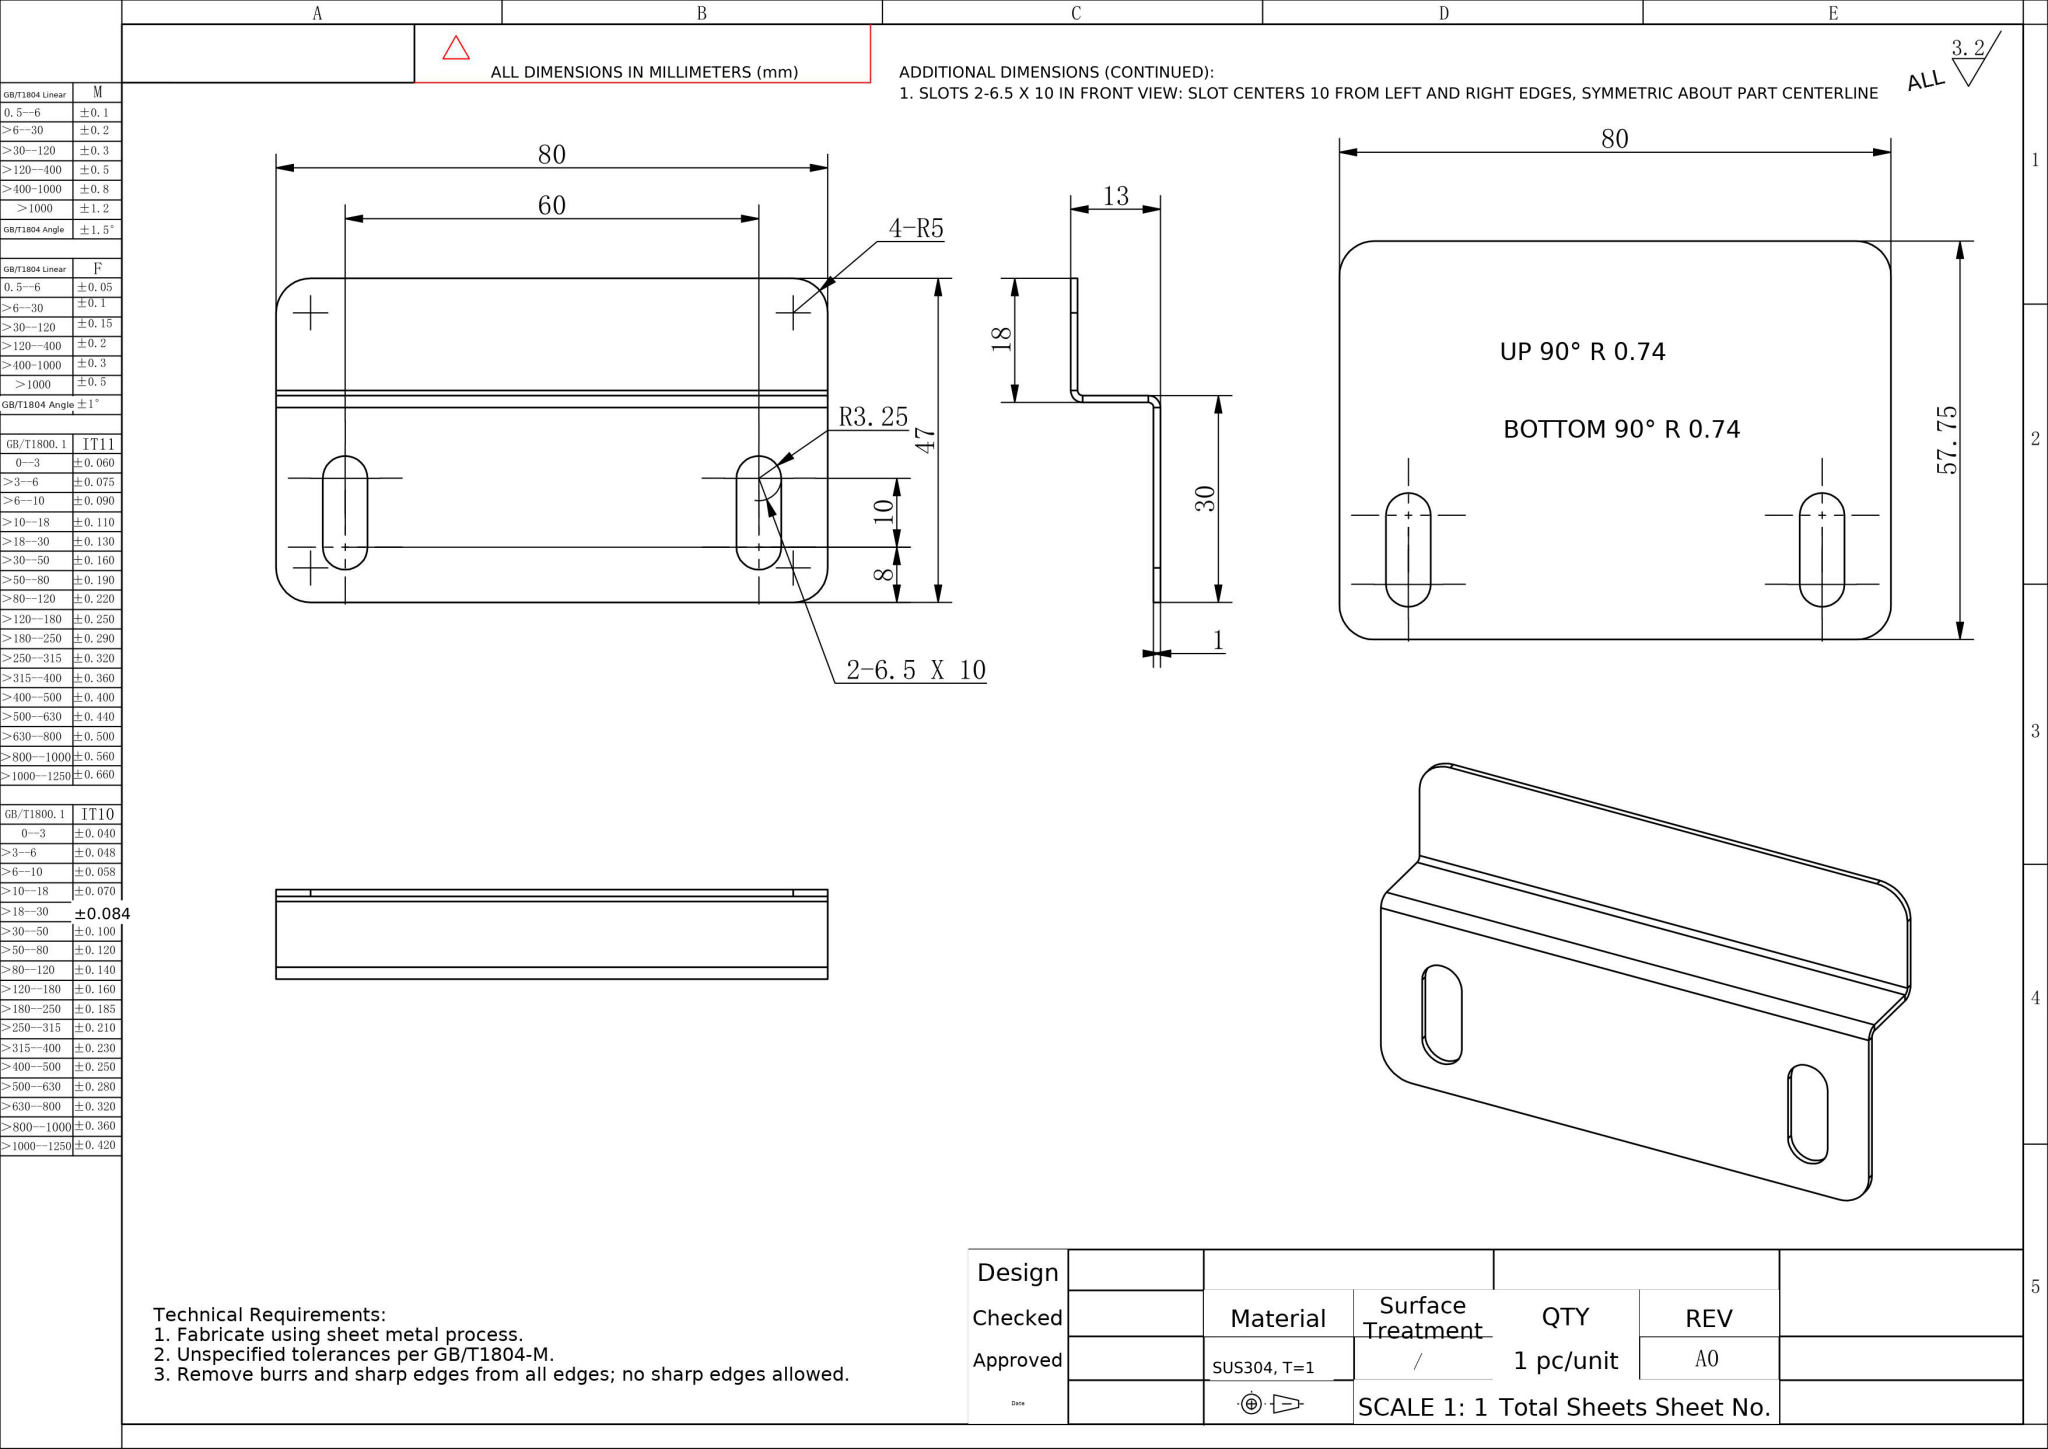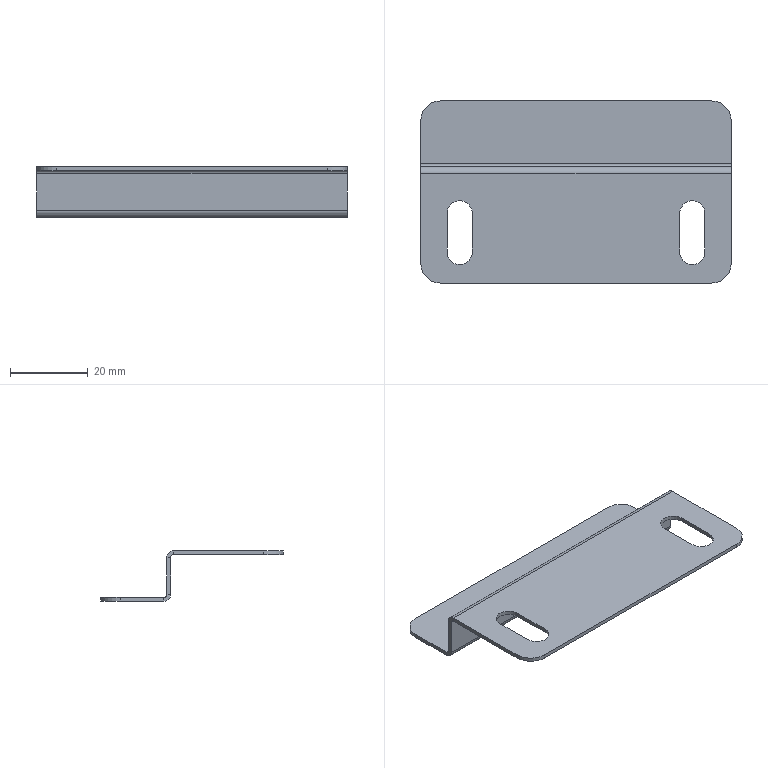Part | NX | mm | 1 solid | 34 faces | box 80 x 47 x 13 mm | volume 4417 mm3 | plane 22 | cylinder 12 | commonest cylinder face diameters 10 x4 6.5 x4 3.473 x2 1.473 x2
STEP:
#1=COLOUR_RGB('',0.7529,0.7529,0.7529);
#2=FILL_AREA_STYLE_COLOUR('',#1);
#3=FILL_AREA_STYLE('',(#2));
#4=SURFACE_STYLE_FILL_AREA(#3);
#5=SURFACE_SIDE_STYLE('',(#4));
#6=SURFACE_STYLE_USAGE(.BOTH.,#5);
#7=PRESENTATION_STYLE_ASSIGNMENT((#6));
#8=CARTESIAN_POINT('',(-40.,-9.737,12.));
#9=VERTEX_POINT('',#8);
#10=CARTESIAN_POINT('',(-40.,-33.,12.));
#11=VERTEX_POINT('',#10);
#12=CARTESIAN_POINT('',(-40.,-0.,12.));
#13=DIRECTION('',(0.,-1.,0.));
#14=VECTOR('',#13,1000.);
#15=LINE('',#12,#14);
#16=EDGE_CURVE('',#9,#11,#15,.T.);
#17=ORIENTED_EDGE('',*,*,#16,.T.);
#18=CARTESIAN_POINT('',(-35.,-38.,12.));
#19=VERTEX_POINT('',#18);
#20=CARTESIAN_POINT('',(-35.,-33.,12.));
#21=DIRECTION('',(0.,0.,1.));
#22=DIRECTION('',(-1.,0.,0.));
#23=AXIS2_PLACEMENT_3D('',#20,#21,#22);
#24=CIRCLE('',#23,5.);
#25=EDGE_CURVE('',#11,#19,#24,.T.);
#26=ORIENTED_EDGE('',*,*,#25,.T.);
#27=CARTESIAN_POINT('',(35.,-38.,12.));
#28=VERTEX_POINT('',#27);
#29=CARTESIAN_POINT('',(0.,-38.,12.));
#30=DIRECTION('',(1.,0.,0.));
#31=VECTOR('',#30,1000.);
#32=LINE('',#29,#31);
#33=EDGE_CURVE('',#19,#28,#32,.T.);
#34=ORIENTED_EDGE('',*,*,#33,.T.);
#35=CARTESIAN_POINT('',(40.,-33.,12.));
#36=VERTEX_POINT('',#35);
#37=CARTESIAN_POINT('',(35.,-33.,12.));
#38=DIRECTION('',(0.,0.,1.));
#39=DIRECTION('',(-1.,0.,0.));
#40=AXIS2_PLACEMENT_3D('',#37,#38,#39);
#41=CIRCLE('',#40,5.);
#42=EDGE_CURVE('',#28,#36,#41,.T.);
#43=ORIENTED_EDGE('',*,*,#42,.T.);
#44=CARTESIAN_POINT('',(40.,-9.737,12.));
#45=VERTEX_POINT('',#44);
#46=CARTESIAN_POINT('',(40.,0.,12.));
#47=DIRECTION('',(0.,1.,0.));
#48=VECTOR('',#47,1000.);
#49=LINE('',#46,#48);
#50=EDGE_CURVE('',#36,#45,#49,.T.);
#51=ORIENTED_EDGE('',*,*,#50,.T.);
#52=CARTESIAN_POINT('',(40.,-9.737,12.));
#53=DIRECTION('',(1.,0.,0.));
#54=VECTOR('',#53,1000.);
#55=LINE('',#52,#54);
#56=EDGE_CURVE('',#9,#45,#55,.T.);
#57=ORIENTED_EDGE('',*,*,#56,.F.);
#58=EDGE_LOOP('',(#17,#26,#34,#43,#51,#57));
#59=FACE_OUTER_BOUND('',#58,.T.);
#60=CARTESIAN_POINT('',(-33.25,-20.,12.));
#61=VERTEX_POINT('',#60);
#62=CARTESIAN_POINT('',(-33.25,-30.,12.));
#63=VERTEX_POINT('',#62);
#64=CARTESIAN_POINT('',(-33.25,-20.,12.));
#65=DIRECTION('',(0.,-1.,0.));
#66=VECTOR('',#65,1000.);
#67=LINE('',#64,#66);
#68=EDGE_CURVE('',#61,#63,#67,.T.);
#69=ORIENTED_EDGE('',*,*,#68,.F.);
#70=CARTESIAN_POINT('',(-26.75,-20.,12.));
#71=VERTEX_POINT('',#70);
#72=CARTESIAN_POINT('',(-30.,-20.,12.));
#73=DIRECTION('',(0.,0.,1.));
#74=DIRECTION('',(1.,0.,0.));
#75=AXIS2_PLACEMENT_3D('',#72,#73,#74);
#76=CIRCLE('',#75,3.25);
#77=EDGE_CURVE('',#71,#61,#76,.T.);
#78=ORIENTED_EDGE('',*,*,#77,.F.);
#79=CARTESIAN_POINT('',(-26.75,-30.,12.));
#80=VERTEX_POINT('',#79);
#81=CARTESIAN_POINT('',(-26.75,-20.,12.));
#82=DIRECTION('',(0.,1.,0.));
#83=VECTOR('',#82,1000.);
#84=LINE('',#81,#83);
#85=EDGE_CURVE('',#80,#71,#84,.T.);
#86=ORIENTED_EDGE('',*,*,#85,.F.);
#87=CARTESIAN_POINT('',(-30.,-30.,12.));
#88=DIRECTION('',(0.,0.,1.));
#89=DIRECTION('',(1.,0.,0.));
#90=AXIS2_PLACEMENT_3D('',#87,#88,#89);
#91=CIRCLE('',#90,3.25);
#92=EDGE_CURVE('',#63,#80,#91,.T.);
#93=ORIENTED_EDGE('',*,*,#92,.F.);
#94=EDGE_LOOP('',(#69,#78,#86,#93));
#95=FACE_BOUND('',#94,.T.);
#96=CARTESIAN_POINT('',(26.75,-20.,12.));
#97=VERTEX_POINT('',#96);
#98=CARTESIAN_POINT('',(33.25,-20.,12.));
#99=VERTEX_POINT('',#98);
#100=CARTESIAN_POINT('',(30.,-20.,12.));
#101=DIRECTION('',(-0.,-0.,-1.));
#102=DIRECTION('',(-1.,0.,0.));
#103=AXIS2_PLACEMENT_3D('',#100,#101,#102);
#104=CIRCLE('',#103,3.25);
#105=EDGE_CURVE('',#97,#99,#104,.T.);
#106=ORIENTED_EDGE('',*,*,#105,.T.);
#107=CARTESIAN_POINT('',(33.25,-30.,12.));
#108=VERTEX_POINT('',#107);
#109=CARTESIAN_POINT('',(33.25,-20.,12.));
#110=DIRECTION('',(-0.,-1.,0.));
#111=VECTOR('',#110,1000.);
#112=LINE('',#109,#111);
#113=EDGE_CURVE('',#99,#108,#112,.T.);
#114=ORIENTED_EDGE('',*,*,#113,.T.);
#115=CARTESIAN_POINT('',(26.75,-30.,12.));
#116=VERTEX_POINT('',#115);
#117=CARTESIAN_POINT('',(30.,-30.,12.));
#118=DIRECTION('',(-0.,-0.,-1.));
#119=DIRECTION('',(-1.,0.,0.));
#120=AXIS2_PLACEMENT_3D('',#117,#118,#119);
#121=CIRCLE('',#120,3.25);
#122=EDGE_CURVE('',#108,#116,#121,.T.);
#123=ORIENTED_EDGE('',*,*,#122,.T.);
#124=CARTESIAN_POINT('',(26.75,-20.,12.));
#125=DIRECTION('',(-0.,1.,0.));
#126=VECTOR('',#125,1000.);
#127=LINE('',#124,#126);
#128=EDGE_CURVE('',#116,#97,#127,.T.);
#129=ORIENTED_EDGE('',*,*,#128,.T.);
#130=EDGE_LOOP('',(#106,#114,#123,#129));
#131=FACE_BOUND('',#130,.T.);
#132=CARTESIAN_POINT('',(0.,0.,12.));
#133=DIRECTION('',(0.,0.,-1.));
#134=DIRECTION('',(-1.,0.,0.));
#135=AXIS2_PLACEMENT_3D('',#132,#133,#134);
#136=PLANE('',#135);
#137=ADVANCED_FACE('',(#59,#95,#131),#136,.F.);
#138=CARTESIAN_POINT('',(-33.25,-20.,11.));
#139=VERTEX_POINT('',#138);
#140=CARTESIAN_POINT('',(-26.75,-20.,11.));
#141=VERTEX_POINT('',#140);
#142=CARTESIAN_POINT('',(-30.,-20.,11.));
#143=DIRECTION('',(0.,0.,-1.));
#144=DIRECTION('',(-1.,0.,0.));
#145=AXIS2_PLACEMENT_3D('',#142,#143,#144);
#146=CIRCLE('',#145,3.25);
#147=EDGE_CURVE('',#139,#141,#146,.T.);
#148=ORIENTED_EDGE('',*,*,#147,.F.);
#149=CARTESIAN_POINT('',(-33.25,-30.,11.));
#150=VERTEX_POINT('',#149);
#151=CARTESIAN_POINT('',(-33.25,-0.,11.));
#152=DIRECTION('',(-0.,1.,0.));
#153=VECTOR('',#152,1000.);
#154=LINE('',#151,#153);
#155=EDGE_CURVE('',#150,#139,#154,.T.);
#156=ORIENTED_EDGE('',*,*,#155,.F.);
#157=CARTESIAN_POINT('',(-26.75,-30.,11.));
#158=VERTEX_POINT('',#157);
#159=CARTESIAN_POINT('',(-30.,-30.,11.));
#160=DIRECTION('',(0.,0.,-1.));
#161=DIRECTION('',(-1.,0.,0.));
#162=AXIS2_PLACEMENT_3D('',#159,#160,#161);
#163=CIRCLE('',#162,3.25);
#164=EDGE_CURVE('',#158,#150,#163,.T.);
#165=ORIENTED_EDGE('',*,*,#164,.F.);
#166=CARTESIAN_POINT('',(-26.75,0.,11.));
#167=DIRECTION('',(0.,-1.,0.));
#168=VECTOR('',#167,1000.);
#169=LINE('',#166,#168);
#170=EDGE_CURVE('',#141,#158,#169,.T.);
#171=ORIENTED_EDGE('',*,*,#170,.F.);
#172=EDGE_LOOP('',(#148,#156,#165,#171));
#173=FACE_BOUND('',#172,.T.);
#174=CARTESIAN_POINT('',(-35.,-38.,11.));
#175=VERTEX_POINT('',#174);
#176=CARTESIAN_POINT('',(35.,-38.,11.));
#177=VERTEX_POINT('',#176);
#178=CARTESIAN_POINT('',(40.,-38.,11.));
#179=DIRECTION('',(1.,0.,0.));
#180=VECTOR('',#179,1000.);
#181=LINE('',#178,#180);
#182=EDGE_CURVE('',#175,#177,#181,.T.);
#183=ORIENTED_EDGE('',*,*,#182,.F.);
#184=CARTESIAN_POINT('',(-40.,-33.,11.));
#185=VERTEX_POINT('',#184);
#186=CARTESIAN_POINT('',(-35.,-33.,11.));
#187=DIRECTION('',(0.,0.,-1.));
#188=DIRECTION('',(-1.,0.,0.));
#189=AXIS2_PLACEMENT_3D('',#186,#187,#188);
#190=CIRCLE('',#189,5.);
#191=EDGE_CURVE('',#175,#185,#190,.T.);
#192=ORIENTED_EDGE('',*,*,#191,.T.);
#193=CARTESIAN_POINT('',(-40.,-9.737,11.));
#194=VERTEX_POINT('',#193);
#195=CARTESIAN_POINT('',(-40.,-38.,11.));
#196=DIRECTION('',(0.,-1.,0.));
#197=VECTOR('',#196,1000.);
#198=LINE('',#195,#197);
#199=EDGE_CURVE('',#194,#185,#198,.T.);
#200=ORIENTED_EDGE('',*,*,#199,.F.);
#201=CARTESIAN_POINT('',(40.,-9.737,11.));
#202=VERTEX_POINT('',#201);
#203=CARTESIAN_POINT('',(40.,-9.737,11.));
#204=DIRECTION('',(-1.,0.,0.));
#205=VECTOR('',#204,1000.);
#206=LINE('',#203,#205);
#207=EDGE_CURVE('',#202,#194,#206,.T.);
#208=ORIENTED_EDGE('',*,*,#207,.F.);
#209=CARTESIAN_POINT('',(40.,-33.,11.));
#210=VERTEX_POINT('',#209);
#211=CARTESIAN_POINT('',(40.,-9.,11.));
#212=DIRECTION('',(0.,1.,0.));
#213=VECTOR('',#212,1000.);
#214=LINE('',#211,#213);
#215=EDGE_CURVE('',#210,#202,#214,.T.);
#216=ORIENTED_EDGE('',*,*,#215,.F.);
#217=CARTESIAN_POINT('',(35.,-33.,11.));
#218=DIRECTION('',(0.,0.,-1.));
#219=DIRECTION('',(-1.,0.,0.));
#220=AXIS2_PLACEMENT_3D('',#217,#218,#219);
#221=CIRCLE('',#220,5.);
#222=EDGE_CURVE('',#210,#177,#221,.T.);
#223=ORIENTED_EDGE('',*,*,#222,.T.);
#224=EDGE_LOOP('',(#183,#192,#200,#208,#216,#223));
#225=FACE_OUTER_BOUND('',#224,.T.);
#226=CARTESIAN_POINT('',(33.25,-30.,11.));
#227=VERTEX_POINT('',#226);
#228=CARTESIAN_POINT('',(33.25,-20.,11.));
#229=VERTEX_POINT('',#228);
#230=CARTESIAN_POINT('',(33.25,-0.,11.));
#231=DIRECTION('',(0.,1.,0.));
#232=VECTOR('',#231,1000.);
#233=LINE('',#230,#232);
#234=EDGE_CURVE('',#227,#229,#233,.T.);
#235=ORIENTED_EDGE('',*,*,#234,.T.);
#236=CARTESIAN_POINT('',(26.75,-20.,11.));
#237=VERTEX_POINT('',#236);
#238=CARTESIAN_POINT('',(30.,-20.,11.));
#239=DIRECTION('',(0.,0.,1.));
#240=DIRECTION('',(-1.,0.,0.));
#241=AXIS2_PLACEMENT_3D('',#238,#239,#240);
#242=CIRCLE('',#241,3.25);
#243=EDGE_CURVE('',#229,#237,#242,.T.);
#244=ORIENTED_EDGE('',*,*,#243,.T.);
#245=CARTESIAN_POINT('',(26.75,-30.,11.));
#246=VERTEX_POINT('',#245);
#247=CARTESIAN_POINT('',(26.75,0.,11.));
#248=DIRECTION('',(0.,-1.,0.));
#249=VECTOR('',#248,1000.);
#250=LINE('',#247,#249);
#251=EDGE_CURVE('',#237,#246,#250,.T.);
#252=ORIENTED_EDGE('',*,*,#251,.T.);
#253=CARTESIAN_POINT('',(30.,-30.,11.));
#254=DIRECTION('',(0.,0.,1.));
#255=DIRECTION('',(-1.,0.,0.));
#256=AXIS2_PLACEMENT_3D('',#253,#254,#255);
#257=CIRCLE('',#256,3.25);
#258=EDGE_CURVE('',#246,#227,#257,.T.);
#259=ORIENTED_EDGE('',*,*,#258,.T.);
#260=EDGE_LOOP('',(#235,#244,#252,#259));
#261=FACE_BOUND('',#260,.T.);
#262=CARTESIAN_POINT('',(0.,0.,11.));
#263=DIRECTION('',(0.,0.,-1.));
#264=DIRECTION('',(-1.,0.,0.));
#265=AXIS2_PLACEMENT_3D('',#262,#263,#264);
#266=PLANE('',#265);
#267=ADVANCED_FACE('',(#173,#225,#261),#266,.T.);
#268=CARTESIAN_POINT('',(-40.,-9.,10.263));
#269=VERTEX_POINT('',#268);
#270=CARTESIAN_POINT('',(-40.,-8.,10.263));
#271=VERTEX_POINT('',#270);
#272=CARTESIAN_POINT('',(-40.,-9.,10.263));
#273=DIRECTION('',(-0.,1.,-0.));
#274=VECTOR('',#273,1000.);
#275=LINE('',#272,#274);
#276=EDGE_CURVE('',#269,#271,#275,.T.);
#277=ORIENTED_EDGE('',*,*,#276,.T.);
#278=CARTESIAN_POINT('',(-40.,-8.,0.7366));
#279=VERTEX_POINT('',#278);
#280=CARTESIAN_POINT('',(-40.,-8.,-0.));
#281=DIRECTION('',(0.,0.,-1.));
#282=VECTOR('',#281,1000.);
#283=LINE('',#280,#282);
#284=EDGE_CURVE('',#271,#279,#283,.T.);
#285=ORIENTED_EDGE('',*,*,#284,.T.);
#286=CARTESIAN_POINT('',(-40.,-9.,0.7366));
#287=VERTEX_POINT('',#286);
#288=CARTESIAN_POINT('',(-40.,-9.,0.7366));
#289=DIRECTION('',(0.,-1.,-0.));
#290=VECTOR('',#289,1000.);
#291=LINE('',#288,#290);
#292=EDGE_CURVE('',#279,#287,#291,.T.);
#293=ORIENTED_EDGE('',*,*,#292,.T.);
#294=CARTESIAN_POINT('',(-40.,-9.,-0.));
#295=DIRECTION('',(0.,0.,-1.));
#296=VECTOR('',#295,1000.);
#297=LINE('',#294,#296);
#298=EDGE_CURVE('',#269,#287,#297,.T.);
#299=ORIENTED_EDGE('',*,*,#298,.F.);
#300=EDGE_LOOP('',(#277,#285,#293,#299));
#301=FACE_OUTER_BOUND('',#300,.T.);
#302=CARTESIAN_POINT('',(-40.,-9.,-0.));
#303=DIRECTION('',(1.,0.,0.));
#304=DIRECTION('',(0.,0.,-1.));
#305=AXIS2_PLACEMENT_3D('',#302,#303,#304);
#306=PLANE('',#305);
#307=ADVANCED_FACE('',(#301),#306,.F.);
#308=CARTESIAN_POINT('',(40.,-9.,10.263));
#309=VERTEX_POINT('',#308);
#310=CARTESIAN_POINT('',(40.,-8.,10.263));
#311=VERTEX_POINT('',#310);
#312=CARTESIAN_POINT('',(40.,-9.,10.263));
#313=DIRECTION('',(0.,1.,-0.));
#314=VECTOR('',#313,1000.);
#315=LINE('',#312,#314);
#316=EDGE_CURVE('',#309,#311,#315,.T.);
#317=ORIENTED_EDGE('',*,*,#316,.F.);
#318=CARTESIAN_POINT('',(40.,-9.,0.7366));
#319=VERTEX_POINT('',#318);
#320=CARTESIAN_POINT('',(40.,-9.,-0.));
#321=DIRECTION('',(0.,-0.,1.));
#322=VECTOR('',#321,1000.);
#323=LINE('',#320,#322);
#324=EDGE_CURVE('',#319,#309,#323,.T.);
#325=ORIENTED_EDGE('',*,*,#324,.F.);
#326=CARTESIAN_POINT('',(40.,-8.,0.7366));
#327=VERTEX_POINT('',#326);
#328=CARTESIAN_POINT('',(40.,-8.,0.7366));
#329=DIRECTION('',(0.,-1.,-0.));
#330=VECTOR('',#329,1000.);
#331=LINE('',#328,#330);
#332=EDGE_CURVE('',#327,#319,#331,.T.);
#333=ORIENTED_EDGE('',*,*,#332,.F.);
#334=CARTESIAN_POINT('',(40.,-8.,12.));
#335=DIRECTION('',(0.,-0.,1.));
#336=VECTOR('',#335,1000.);
#337=LINE('',#334,#336);
#338=EDGE_CURVE('',#327,#311,#337,.T.);
#339=ORIENTED_EDGE('',*,*,#338,.T.);
#340=EDGE_LOOP('',(#317,#325,#333,#339));
#341=FACE_OUTER_BOUND('',#340,.T.);
#342=CARTESIAN_POINT('',(40.,-9.,12.));
#343=DIRECTION('',(-1.,-0.,0.));
#344=DIRECTION('',(0.,0.,1.));
#345=AXIS2_PLACEMENT_3D('',#342,#343,#344);
#346=PLANE('',#345);
#347=ADVANCED_FACE('',(#341),#346,.F.);
#348=CARTESIAN_POINT('',(-40.,-9.,10.263));
#349=DIRECTION('',(1.,0.,-0.));
#350=VECTOR('',#349,1000.);
#351=LINE('',#348,#350);
#352=EDGE_CURVE('',#269,#309,#351,.T.);
#353=ORIENTED_EDGE('',*,*,#352,.F.);
#354=ORIENTED_EDGE('',*,*,#298,.T.);
#355=CARTESIAN_POINT('',(-40.,-9.,0.7366));
#356=DIRECTION('',(-1.,0.,0.));
#357=VECTOR('',#356,1000.);
#358=LINE('',#355,#357);
#359=EDGE_CURVE('',#319,#287,#358,.T.);
#360=ORIENTED_EDGE('',*,*,#359,.F.);
#361=ORIENTED_EDGE('',*,*,#324,.T.);
#362=EDGE_LOOP('',(#353,#354,#360,#361));
#363=FACE_OUTER_BOUND('',#362,.T.);
#364=CARTESIAN_POINT('',(0.,-9.,-0.));
#365=DIRECTION('',(0.,1.,0.));
#366=DIRECTION('',(0.,-0.,1.));
#367=AXIS2_PLACEMENT_3D('',#364,#365,#366);
#368=PLANE('',#367);
#369=ADVANCED_FACE('',(#363),#368,.F.);
#370=ORIENTED_EDGE('',*,*,#284,.F.);
#371=CARTESIAN_POINT('',(-40.,-8.,10.263));
#372=DIRECTION('',(1.,0.,-0.));
#373=VECTOR('',#372,1000.);
#374=LINE('',#371,#373);
#375=EDGE_CURVE('',#271,#311,#374,.T.);
#376=ORIENTED_EDGE('',*,*,#375,.T.);
#377=ORIENTED_EDGE('',*,*,#338,.F.);
#378=CARTESIAN_POINT('',(-40.,-8.,0.7366));
#379=DIRECTION('',(1.,0.,0.));
#380=VECTOR('',#379,1000.);
#381=LINE('',#378,#380);
#382=EDGE_CURVE('',#279,#327,#381,.T.);
#383=ORIENTED_EDGE('',*,*,#382,.F.);
#384=EDGE_LOOP('',(#370,#376,#377,#383));
#385=FACE_OUTER_BOUND('',#384,.T.);
#386=CARTESIAN_POINT('',(0.,-8.,-0.));
#387=DIRECTION('',(0.,1.,0.));
#388=DIRECTION('',(0.,-0.,1.));
#389=AXIS2_PLACEMENT_3D('',#386,#387,#388);
#390=PLANE('',#389);
#391=ADVANCED_FACE('',(#385),#390,.T.);
#392=CARTESIAN_POINT('',(40.,-7.263,-1.));
#393=VERTEX_POINT('',#392);
#394=CARTESIAN_POINT('',(40.,4.,-1.));
#395=VERTEX_POINT('',#394);
#396=CARTESIAN_POINT('',(40.,9.,-1.));
#397=DIRECTION('',(0.,1.,0.));
#398=VECTOR('',#397,1000.);
#399=LINE('',#396,#398);
#400=EDGE_CURVE('',#393,#395,#399,.T.);
#401=ORIENTED_EDGE('',*,*,#400,.T.);
#402=CARTESIAN_POINT('',(40.,4.,0.));
#403=VERTEX_POINT('',#402);
#404=CARTESIAN_POINT('',(40.,4.,-1.));
#405=DIRECTION('',(0.,0.,1.));
#406=VECTOR('',#405,1000.);
#407=LINE('',#404,#406);
#408=EDGE_CURVE('',#395,#403,#407,.T.);
#409=ORIENTED_EDGE('',*,*,#408,.T.);
#410=CARTESIAN_POINT('',(40.,-7.263,0.));
#411=VERTEX_POINT('',#410);
#412=CARTESIAN_POINT('',(40.,9.,0.));
#413=DIRECTION('',(0.,1.,0.));
#414=VECTOR('',#413,1000.);
#415=LINE('',#412,#414);
#416=EDGE_CURVE('',#411,#403,#415,.T.);
#417=ORIENTED_EDGE('',*,*,#416,.F.);
#418=CARTESIAN_POINT('',(40.,-7.263,-0.));
#419=DIRECTION('',(0.,0.,-1.));
#420=VECTOR('',#419,1000.);
#421=LINE('',#418,#420);
#422=EDGE_CURVE('',#411,#393,#421,.T.);
#423=ORIENTED_EDGE('',*,*,#422,.T.);
#424=EDGE_LOOP('',(#401,#409,#417,#423));
#425=FACE_OUTER_BOUND('',#424,.T.);
#426=CARTESIAN_POINT('',(40.,9.,-1.));
#427=DIRECTION('',(1.,0.,0.));
#428=DIRECTION('',(0.,0.,-1.));
#429=AXIS2_PLACEMENT_3D('',#426,#427,#428);
#430=PLANE('',#429);
#431=ADVANCED_FACE('',(#425),#430,.T.);
#432=CARTESIAN_POINT('',(35.,9.,-1.));
#433=VERTEX_POINT('',#432);
#434=CARTESIAN_POINT('',(-35.,9.,-1.));
#435=VERTEX_POINT('',#434);
#436=CARTESIAN_POINT('',(-40.,9.,-1.));
#437=DIRECTION('',(-1.,0.,0.));
#438=VECTOR('',#437,1000.);
#439=LINE('',#436,#438);
#440=EDGE_CURVE('',#433,#435,#439,.T.);
#441=ORIENTED_EDGE('',*,*,#440,.F.);
#442=CARTESIAN_POINT('',(35.,4.,-1.));
#443=DIRECTION('',(0.,0.,-1.));
#444=DIRECTION('',(1.,0.,0.));
#445=AXIS2_PLACEMENT_3D('',#442,#443,#444);
#446=CIRCLE('',#445,5.);
#447=EDGE_CURVE('',#433,#395,#446,.T.);
#448=ORIENTED_EDGE('',*,*,#447,.T.);
#449=ORIENTED_EDGE('',*,*,#400,.F.);
#450=CARTESIAN_POINT('',(-40.,-7.263,-1.));
#451=VERTEX_POINT('',#450);
#452=CARTESIAN_POINT('',(40.,-7.263,-1.));
#453=DIRECTION('',(-1.,0.,0.));
#454=VECTOR('',#453,1000.);
#455=LINE('',#452,#454);
#456=EDGE_CURVE('',#393,#451,#455,.T.);
#457=ORIENTED_EDGE('',*,*,#456,.T.);
#458=CARTESIAN_POINT('',(-40.,4.,-1.));
#459=VERTEX_POINT('',#458);
#460=CARTESIAN_POINT('',(-40.,9.,-1.));
#461=DIRECTION('',(0.,-1.,0.));
#462=VECTOR('',#461,1000.);
#463=LINE('',#460,#462);
#464=EDGE_CURVE('',#459,#451,#463,.T.);
#465=ORIENTED_EDGE('',*,*,#464,.F.);
#466=CARTESIAN_POINT('',(-35.,4.,-1.));
#467=DIRECTION('',(0.,0.,-1.));
#468=DIRECTION('',(1.,0.,0.));
#469=AXIS2_PLACEMENT_3D('',#466,#467,#468);
#470=CIRCLE('',#469,5.);
#471=EDGE_CURVE('',#459,#435,#470,.T.);
#472=ORIENTED_EDGE('',*,*,#471,.T.);
#473=EDGE_LOOP('',(#441,#448,#449,#457,#465,#472));
#474=FACE_OUTER_BOUND('',#473,.T.);
#475=CARTESIAN_POINT('',(0.,0.,-1.));
#476=DIRECTION('',(0.,0.,1.));
#477=DIRECTION('',(1.,0.,0.));
#478=AXIS2_PLACEMENT_3D('',#475,#476,#477);
#479=PLANE('',#478);
#480=ADVANCED_FACE('',(#474),#479,.F.);
#481=ORIENTED_EDGE('',*,*,#416,.T.);
#482=CARTESIAN_POINT('',(35.,9.,0.));
#483=VERTEX_POINT('',#482);
#484=CARTESIAN_POINT('',(35.,4.,0.));
#485=DIRECTION('',(0.,0.,1.));
#486=DIRECTION('',(1.,0.,0.));
#487=AXIS2_PLACEMENT_3D('',#484,#485,#486);
#488=CIRCLE('',#487,5.);
#489=EDGE_CURVE('',#403,#483,#488,.T.);
#490=ORIENTED_EDGE('',*,*,#489,.T.);
#491=CARTESIAN_POINT('',(-35.,9.,0.));
#492=VERTEX_POINT('',#491);
#493=CARTESIAN_POINT('',(-40.,9.,0.));
#494=DIRECTION('',(-1.,0.,0.));
#495=VECTOR('',#494,1000.);
#496=LINE('',#493,#495);
#497=EDGE_CURVE('',#483,#492,#496,.T.);
#498=ORIENTED_EDGE('',*,*,#497,.T.);
#499=CARTESIAN_POINT('',(-40.,4.,0.));
#500=VERTEX_POINT('',#499);
#501=CARTESIAN_POINT('',(-35.,4.,0.));
#502=DIRECTION('',(0.,0.,1.));
#503=DIRECTION('',(1.,0.,0.));
#504=AXIS2_PLACEMENT_3D('',#501,#502,#503);
#505=CIRCLE('',#504,5.);
#506=EDGE_CURVE('',#492,#500,#505,.T.);
#507=ORIENTED_EDGE('',*,*,#506,.T.);
#508=CARTESIAN_POINT('',(-40.,-7.263,-0.));
#509=VERTEX_POINT('',#508);
#510=CARTESIAN_POINT('',(-40.,9.,0.));
#511=DIRECTION('',(0.,-1.,0.));
#512=VECTOR('',#511,1000.);
#513=LINE('',#510,#512);
#514=EDGE_CURVE('',#500,#509,#513,.T.);
#515=ORIENTED_EDGE('',*,*,#514,.T.);
#516=CARTESIAN_POINT('',(40.,-7.263,-0.));
#517=DIRECTION('',(-1.,0.,0.));
#518=VECTOR('',#517,1000.);
#519=LINE('',#516,#518);
#520=EDGE_CURVE('',#411,#509,#519,.T.);
#521=ORIENTED_EDGE('',*,*,#520,.F.);
#522=EDGE_LOOP('',(#481,#490,#498,#507,#515,#521));
#523=FACE_OUTER_BOUND('',#522,.T.);
#524=CARTESIAN_POINT('',(0.,0.,0.));
#525=DIRECTION('',(0.,0.,1.));
#526=DIRECTION('',(1.,0.,0.));
#527=AXIS2_PLACEMENT_3D('',#524,#525,#526);
#528=PLANE('',#527);
#529=ADVANCED_FACE('',(#523),#528,.T.);
#530=ORIENTED_EDGE('',*,*,#514,.F.);
#531=CARTESIAN_POINT('',(-40.,4.,-1.));
#532=DIRECTION('',(0.,0.,-1.));
#533=VECTOR('',#532,1000.);
#534=LINE('',#531,#533);
#535=EDGE_CURVE('',#500,#459,#534,.T.);
#536=ORIENTED_EDGE('',*,*,#535,.T.);
#537=ORIENTED_EDGE('',*,*,#464,.T.);
#538=CARTESIAN_POINT('',(-40.,-7.263,-0.));
#539=DIRECTION('',(0.,0.,-1.));
#540=VECTOR('',#539,1000.);
#541=LINE('',#538,#540);
#542=EDGE_CURVE('',#509,#451,#541,.T.);
#543=ORIENTED_EDGE('',*,*,#542,.F.);
#544=EDGE_LOOP('',(#530,#536,#537,#543));
#545=FACE_OUTER_BOUND('',#544,.T.);
#546=CARTESIAN_POINT('',(-40.,9.,-1.));
#547=DIRECTION('',(-1.,0.,0.));
#548=DIRECTION('',(0.,0.,1.));
#549=AXIS2_PLACEMENT_3D('',#546,#547,#548);
#550=PLANE('',#549);
#551=ADVANCED_FACE('',(#545),#550,.T.);
#552=ORIENTED_EDGE('',*,*,#497,.F.);
#553=CARTESIAN_POINT('',(35.,9.,-1.));
#554=DIRECTION('',(0.,0.,-1.));
#555=VECTOR('',#554,1000.);
#556=LINE('',#553,#555);
#557=EDGE_CURVE('',#483,#433,#556,.T.);
#558=ORIENTED_EDGE('',*,*,#557,.T.);
#559=ORIENTED_EDGE('',*,*,#440,.T.);
#560=CARTESIAN_POINT('',(-35.,9.,-1.));
#561=DIRECTION('',(0.,0.,1.));
#562=VECTOR('',#561,1000.);
#563=LINE('',#560,#562);
#564=EDGE_CURVE('',#435,#492,#563,.T.);
#565=ORIENTED_EDGE('',*,*,#564,.T.);
#566=EDGE_LOOP('',(#552,#558,#559,#565));
#567=FACE_OUTER_BOUND('',#566,.T.);
#568=CARTESIAN_POINT('',(-40.,9.,-1.));
#569=DIRECTION('',(0.,1.,0.));
#570=DIRECTION('',(0.,0.,1.));
#571=AXIS2_PLACEMENT_3D('',#568,#569,#570);
#572=PLANE('',#571);
#573=ADVANCED_FACE('',(#567),#572,.T.);
#574=ORIENTED_EDGE('',*,*,#292,.F.);
#575=CARTESIAN_POINT('',(-40.,-7.263,0.7366));
#576=DIRECTION('',(-1.,0.,0.));
#577=DIRECTION('',(0.,0.,-1.));
#578=AXIS2_PLACEMENT_3D('',#575,#576,#577);
#579=CIRCLE('',#578,0.7366);
#580=EDGE_CURVE('',#509,#279,#579,.T.);
#581=ORIENTED_EDGE('',*,*,#580,.F.);
#582=ORIENTED_EDGE('',*,*,#542,.T.);
#583=CARTESIAN_POINT('',(-40.,-7.263,0.7366));
#584=DIRECTION('',(-1.,0.,0.));
#585=DIRECTION('',(0.,0.,-1.));
#586=AXIS2_PLACEMENT_3D('',#583,#584,#585);
#587=CIRCLE('',#586,1.737);
#588=EDGE_CURVE('',#451,#287,#587,.T.);
#589=ORIENTED_EDGE('',*,*,#588,.T.);
#590=EDGE_LOOP('',(#574,#581,#582,#589));
#591=FACE_OUTER_BOUND('',#590,.T.);
#592=CARTESIAN_POINT('',(-40.,-7.263,0.7366));
#593=DIRECTION('',(-1.,0.,0.));
#594=DIRECTION('',(0.,0.,1.));
#595=AXIS2_PLACEMENT_3D('',#592,#593,#594);
#596=PLANE('',#595);
#597=ADVANCED_FACE('',(#591),#596,.T.);
#598=CARTESIAN_POINT('',(40.,-7.263,0.7366));
#599=DIRECTION('',(1.,0.,0.));
#600=DIRECTION('',(0.,0.,-1.));
#601=AXIS2_PLACEMENT_3D('',#598,#599,#600);
#602=CIRCLE('',#601,0.7366);
#603=EDGE_CURVE('',#327,#411,#602,.T.);
#604=ORIENTED_EDGE('',*,*,#603,.F.);
#605=ORIENTED_EDGE('',*,*,#332,.T.);
#606=CARTESIAN_POINT('',(40.,-7.263,0.7366));
#607=DIRECTION('',(1.,0.,0.));
#608=DIRECTION('',(0.,0.,-1.));
#609=AXIS2_PLACEMENT_3D('',#606,#607,#608);
#610=CIRCLE('',#609,1.737);
#611=EDGE_CURVE('',#319,#393,#610,.T.);
#612=ORIENTED_EDGE('',*,*,#611,.T.);
#613=ORIENTED_EDGE('',*,*,#422,.F.);
#614=EDGE_LOOP('',(#604,#605,#612,#613));
#615=FACE_OUTER_BOUND('',#614,.T.);
#616=CARTESIAN_POINT('',(40.,-7.263,0.7366));
#617=DIRECTION('',(-1.,0.,0.));
#618=DIRECTION('',(0.,0.,1.));
#619=AXIS2_PLACEMENT_3D('',#616,#617,#618);
#620=PLANE('',#619);
#621=ADVANCED_FACE('',(#615),#620,.F.);
#622=ORIENTED_EDGE('',*,*,#456,.F.);
#623=ORIENTED_EDGE('',*,*,#611,.F.);
#624=ORIENTED_EDGE('',*,*,#359,.T.);
#625=ORIENTED_EDGE('',*,*,#588,.F.);
#626=EDGE_LOOP('',(#622,#623,#624,#625));
#627=FACE_OUTER_BOUND('',#626,.T.);
#628=CARTESIAN_POINT('',(40.,-7.263,0.7366));
#629=DIRECTION('',(1.,0.,0.));
#630=DIRECTION('',(0.,-1.,-0.));
#631=AXIS2_PLACEMENT_3D('',#628,#629,#630);
#632=CYLINDRICAL_SURFACE('',#631,1.737);
#633=ADVANCED_FACE('',(#627),#632,.T.);
#634=ORIENTED_EDGE('',*,*,#520,.T.);
#635=ORIENTED_EDGE('',*,*,#580,.T.);
#636=ORIENTED_EDGE('',*,*,#382,.T.);
#637=ORIENTED_EDGE('',*,*,#603,.T.);
#638=EDGE_LOOP('',(#634,#635,#636,#637));
#639=FACE_OUTER_BOUND('',#638,.T.);
#640=CARTESIAN_POINT('',(40.,-7.263,0.7366));
#641=DIRECTION('',(1.,0.,0.));
#642=DIRECTION('',(0.,-1.,-0.));
#643=AXIS2_PLACEMENT_3D('',#640,#641,#642);
#644=CYLINDRICAL_SURFACE('',#643,0.7366);
#645=ADVANCED_FACE('',(#639),#644,.F.);
#646=CARTESIAN_POINT('',(40.,-9.737,12.));
#647=DIRECTION('',(0.,0.,1.));
#648=VECTOR('',#647,1000.);
#649=LINE('',#646,#648);
#650=EDGE_CURVE('',#202,#45,#649,.T.);
#651=ORIENTED_EDGE('',*,*,#650,.F.);
#652=CARTESIAN_POINT('',(40.,-9.737,10.263));
#653=DIRECTION('',(1.,0.,-0.));
#654=DIRECTION('',(0.,0.,1.));
#655=AXIS2_PLACEMENT_3D('',#652,#653,#654);
#656=CIRCLE('',#655,0.7366);
#657=EDGE_CURVE('',#309,#202,#656,.T.);
#658=ORIENTED_EDGE('',*,*,#657,.F.);
#659=ORIENTED_EDGE('',*,*,#316,.T.);
#660=CARTESIAN_POINT('',(40.,-9.737,10.263));
#661=DIRECTION('',(1.,0.,-0.));
#662=DIRECTION('',(0.,0.,1.));
#663=AXIS2_PLACEMENT_3D('',#660,#661,#662);
#664=CIRCLE('',#663,1.737);
#665=EDGE_CURVE('',#311,#45,#664,.T.);
#666=ORIENTED_EDGE('',*,*,#665,.T.);
#667=EDGE_LOOP('',(#651,#658,#659,#666));
#668=FACE_OUTER_BOUND('',#667,.T.);
#669=CARTESIAN_POINT('',(40.,-9.737,10.263));
#670=DIRECTION('',(1.,0.,-0.));
#671=DIRECTION('',(-0.,0.,-1.));
#672=AXIS2_PLACEMENT_3D('',#669,#670,#671);
#673=PLANE('',#672);
#674=ADVANCED_FACE('',(#668),#673,.T.);
#675=CARTESIAN_POINT('',(-40.,-9.737,10.263));
#676=DIRECTION('',(-1.,0.,0.));
#677=DIRECTION('',(0.,0.,1.));
#678=AXIS2_PLACEMENT_3D('',#675,#676,#677);
#679=CIRCLE('',#678,0.7366);
#680=EDGE_CURVE('',#194,#269,#679,.T.);
#681=ORIENTED_EDGE('',*,*,#680,.F.);
#682=CARTESIAN_POINT('',(-40.,-9.737,11.));
#683=DIRECTION('',(0.,0.,1.));
#684=VECTOR('',#683,1000.);
#685=LINE('',#682,#684);
#686=EDGE_CURVE('',#194,#9,#685,.T.);
#687=ORIENTED_EDGE('',*,*,#686,.T.);
#688=CARTESIAN_POINT('',(-40.,-9.737,10.263));
#689=DIRECTION('',(-1.,0.,0.));
#690=DIRECTION('',(0.,0.,1.));
#691=AXIS2_PLACEMENT_3D('',#688,#689,#690);
#692=CIRCLE('',#691,1.737);
#693=EDGE_CURVE('',#9,#271,#692,.T.);
#694=ORIENTED_EDGE('',*,*,#693,.T.);
#695=ORIENTED_EDGE('',*,*,#276,.F.);
#696=EDGE_LOOP('',(#681,#687,#694,#695));
#697=FACE_OUTER_BOUND('',#696,.T.);
#698=CARTESIAN_POINT('',(-40.,-9.737,10.263));
#699=DIRECTION('',(1.,0.,-0.));
#700=DIRECTION('',(-0.,0.,-1.));
#701=AXIS2_PLACEMENT_3D('',#698,#699,#700);
#702=PLANE('',#701);
#703=ADVANCED_FACE('',(#697),#702,.F.);
#704=ORIENTED_EDGE('',*,*,#375,.F.);
#705=ORIENTED_EDGE('',*,*,#693,.F.);
#706=ORIENTED_EDGE('',*,*,#56,.T.);
#707=ORIENTED_EDGE('',*,*,#665,.F.);
#708=EDGE_LOOP('',(#704,#705,#706,#707));
#709=FACE_OUTER_BOUND('',#708,.T.);
#710=CARTESIAN_POINT('',(-40.,-9.737,10.263));
#711=DIRECTION('',(-1.,0.,0.));
#712=DIRECTION('',(0.,0.,1.));
#713=AXIS2_PLACEMENT_3D('',#710,#711,#712);
#714=CYLINDRICAL_SURFACE('',#713,1.737);
#715=ADVANCED_FACE('',(#709),#714,.T.);
#716=ORIENTED_EDGE('',*,*,#352,.T.);
#717=ORIENTED_EDGE('',*,*,#657,.T.);
#718=ORIENTED_EDGE('',*,*,#207,.T.);
#719=ORIENTED_EDGE('',*,*,#680,.T.);
#720=EDGE_LOOP('',(#716,#717,#718,#719));
#721=FACE_OUTER_BOUND('',#720,.T.);
#722=CARTESIAN_POINT('',(-40.,-9.737,10.263));
#723=DIRECTION('',(-1.,0.,0.));
#724=DIRECTION('',(0.,0.,1.));
#725=AXIS2_PLACEMENT_3D('',#722,#723,#724);
#726=CYLINDRICAL_SURFACE('',#725,0.7366);
#727=ADVANCED_FACE('',(#721),#726,.F.);
#728=ORIENTED_EDGE('',*,*,#50,.F.);
#729=CARTESIAN_POINT('',(40.,-33.,12.));
#730=DIRECTION('',(0.,-0.,-1.));
#731=VECTOR('',#730,1000.);
#732=LINE('',#729,#731);
#733=EDGE_CURVE('',#36,#210,#732,.T.);
#734=ORIENTED_EDGE('',*,*,#733,.T.);
#735=ORIENTED_EDGE('',*,*,#215,.T.);
#736=ORIENTED_EDGE('',*,*,#650,.T.);
#737=EDGE_LOOP('',(#728,#734,#735,#736));
#738=FACE_OUTER_BOUND('',#737,.T.);
#739=CARTESIAN_POINT('',(40.,-9.,12.));
#740=DIRECTION('',(-1.,0.,0.));
#741=DIRECTION('',(0.,0.,1.));
#742=AXIS2_PLACEMENT_3D('',#739,#740,#741);
#743=PLANE('',#742);
#744=ADVANCED_FACE('',(#738),#743,.F.);
#745=ORIENTED_EDGE('',*,*,#199,.T.);
#746=CARTESIAN_POINT('',(-40.,-33.,12.));
#747=DIRECTION('',(-0.,0.,1.));
#748=VECTOR('',#747,1000.);
#749=LINE('',#746,#748);
#750=EDGE_CURVE('',#185,#11,#749,.T.);
#751=ORIENTED_EDGE('',*,*,#750,.T.);
#752=ORIENTED_EDGE('',*,*,#16,.F.);
#753=ORIENTED_EDGE('',*,*,#686,.F.);
#754=EDGE_LOOP('',(#745,#751,#752,#753));
#755=FACE_OUTER_BOUND('',#754,.T.);
#756=CARTESIAN_POINT('',(-40.,-38.,12.));
#757=DIRECTION('',(1.,0.,-0.));
#758=DIRECTION('',(-0.,1.,0.));
#759=AXIS2_PLACEMENT_3D('',#756,#757,#758);
#760=PLANE('',#759);
#761=ADVANCED_FACE('',(#755),#760,.F.);
#762=ORIENTED_EDGE('',*,*,#33,.F.);
#763=CARTESIAN_POINT('',(-35.,-38.,12.));
#764=DIRECTION('',(0.,-0.,-1.));
#765=VECTOR('',#764,1000.);
#766=LINE('',#763,#765);
#767=EDGE_CURVE('',#19,#175,#766,.T.);
#768=ORIENTED_EDGE('',*,*,#767,.T.);
#769=ORIENTED_EDGE('',*,*,#182,.T.);
#770=CARTESIAN_POINT('',(35.,-38.,12.));
#771=DIRECTION('',(0.,0.,1.));
#772=VECTOR('',#771,1000.);
#773=LINE('',#770,#772);
#774=EDGE_CURVE('',#177,#28,#773,.T.);
#775=ORIENTED_EDGE('',*,*,#774,.T.);
#776=EDGE_LOOP('',(#762,#768,#769,#775));
#777=FACE_OUTER_BOUND('',#776,.T.);
#778=CARTESIAN_POINT('',(40.,-38.,12.));
#779=DIRECTION('',(0.,1.,-0.));
#780=DIRECTION('',(0.,0.,1.));
#781=AXIS2_PLACEMENT_3D('',#778,#779,#780);
#782=PLANE('',#781);
#783=ADVANCED_FACE('',(#777),#782,.F.);
#784=ORIENTED_EDGE('',*,*,#25,.F.);
#785=ORIENTED_EDGE('',*,*,#750,.F.);
#786=ORIENTED_EDGE('',*,*,#191,.F.);
#787=ORIENTED_EDGE('',*,*,#767,.F.);
#788=EDGE_LOOP('',(#784,#785,#786,#787));
#789=FACE_OUTER_BOUND('',#788,.T.);
#790=CARTESIAN_POINT('',(-35.,-33.,12.));
#791=DIRECTION('',(0.,-0.,-1.));
#792=DIRECTION('',(0.,1.,0.));
#793=AXIS2_PLACEMENT_3D('',#790,#791,#792);
#794=CYLINDRICAL_SURFACE('',#793,5.);
#795=ADVANCED_FACE('',(#789),#794,.T.);
#796=ORIENTED_EDGE('',*,*,#42,.F.);
#797=ORIENTED_EDGE('',*,*,#774,.F.);
#798=ORIENTED_EDGE('',*,*,#222,.F.);
#799=ORIENTED_EDGE('',*,*,#733,.F.);
#800=EDGE_LOOP('',(#796,#797,#798,#799));
#801=FACE_OUTER_BOUND('',#800,.T.);
#802=CARTESIAN_POINT('',(35.,-33.,12.));
#803=DIRECTION('',(0.,-0.,-1.));
#804=DIRECTION('',(0.,1.,0.));
#805=AXIS2_PLACEMENT_3D('',#802,#803,#804);
#806=CYLINDRICAL_SURFACE('',#805,5.);
#807=ADVANCED_FACE('',(#801),#806,.T.);
#808=ORIENTED_EDGE('',*,*,#447,.F.);
#809=ORIENTED_EDGE('',*,*,#557,.F.);
#810=ORIENTED_EDGE('',*,*,#489,.F.);
#811=ORIENTED_EDGE('',*,*,#408,.F.);
#812=EDGE_LOOP('',(#808,#809,#810,#811));
#813=FACE_OUTER_BOUND('',#812,.T.);
#814=CARTESIAN_POINT('',(35.,4.,-1.));
#815=DIRECTION('',(0.,0.,1.));
#816=DIRECTION('',(1.,0.,0.));
#817=AXIS2_PLACEMENT_3D('',#814,#815,#816);
#818=CYLINDRICAL_SURFACE('',#817,5.);
#819=ADVANCED_FACE('',(#813),#818,.T.);
#820=ORIENTED_EDGE('',*,*,#471,.F.);
#821=ORIENTED_EDGE('',*,*,#535,.F.);
#822=ORIENTED_EDGE('',*,*,#506,.F.);
#823=ORIENTED_EDGE('',*,*,#564,.F.);
#824=EDGE_LOOP('',(#820,#821,#822,#823));
#825=FACE_OUTER_BOUND('',#824,.T.);
#826=CARTESIAN_POINT('',(-35.,4.,-1.));
#827=DIRECTION('',(0.,0.,1.));
#828=DIRECTION('',(1.,0.,0.));
#829=AXIS2_PLACEMENT_3D('',#826,#827,#828);
#830=CYLINDRICAL_SURFACE('',#829,5.);
#831=ADVANCED_FACE('',(#825),#830,.T.);
#832=ORIENTED_EDGE('',*,*,#147,.T.);
#833=CARTESIAN_POINT('',(-26.75,-20.,2.));
#834=DIRECTION('',(0.,0.,1.));
#835=VECTOR('',#834,1000.);
#836=LINE('',#833,#835);
#837=EDGE_CURVE('',#141,#71,#836,.T.);
#838=ORIENTED_EDGE('',*,*,#837,.T.);
#839=ORIENTED_EDGE('',*,*,#77,.T.);
#840=CARTESIAN_POINT('',(-33.25,-20.,2.));
#841=DIRECTION('',(0.,0.,1.));
#842=VECTOR('',#841,1000.);
#843=LINE('',#840,#842);
#844=EDGE_CURVE('',#139,#61,#843,.T.);
#845=ORIENTED_EDGE('',*,*,#844,.F.);
#846=EDGE_LOOP('',(#832,#838,#839,#845));
#847=FACE_OUTER_BOUND('',#846,.T.);
#848=CARTESIAN_POINT('',(-30.,-20.,2.));
#849=DIRECTION('',(0.,0.,1.));
#850=DIRECTION('',(1.,0.,0.));
#851=AXIS2_PLACEMENT_3D('',#848,#849,#850);
#852=CYLINDRICAL_SURFACE('',#851,3.25);
#853=ADVANCED_FACE('',(#847),#852,.F.);
#854=ORIENTED_EDGE('',*,*,#170,.T.);
#855=CARTESIAN_POINT('',(-26.75,-30.,2.));
#856=DIRECTION('',(0.,0.,1.));
#857=VECTOR('',#856,1000.);
#858=LINE('',#855,#857);
#859=EDGE_CURVE('',#158,#80,#858,.T.);
#860=ORIENTED_EDGE('',*,*,#859,.T.);
#861=ORIENTED_EDGE('',*,*,#85,.T.);
#862=ORIENTED_EDGE('',*,*,#837,.F.);
#863=EDGE_LOOP('',(#854,#860,#861,#862));
#864=FACE_OUTER_BOUND('',#863,.T.);
#865=CARTESIAN_POINT('',(-26.75,-20.,2.));
#866=DIRECTION('',(1.,0.,0.));
#867=DIRECTION('',(0.,0.,-1.));
#868=AXIS2_PLACEMENT_3D('',#865,#866,#867);
#869=PLANE('',#868);
#870=ADVANCED_FACE('',(#864),#869,.F.);
#871=ORIENTED_EDGE('',*,*,#164,.T.);
#872=CARTESIAN_POINT('',(-33.25,-30.,2.));
#873=DIRECTION('',(0.,0.,1.));
#874=VECTOR('',#873,1000.);
#875=LINE('',#872,#874);
#876=EDGE_CURVE('',#150,#63,#875,.T.);
#877=ORIENTED_EDGE('',*,*,#876,.T.);
#878=ORIENTED_EDGE('',*,*,#92,.T.);
#879=ORIENTED_EDGE('',*,*,#859,.F.);
#880=EDGE_LOOP('',(#871,#877,#878,#879));
#881=FACE_OUTER_BOUND('',#880,.T.);
#882=CARTESIAN_POINT('',(-30.,-30.,2.));
#883=DIRECTION('',(0.,0.,1.));
#884=DIRECTION('',(1.,0.,0.));
#885=AXIS2_PLACEMENT_3D('',#882,#883,#884);
#886=CYLINDRICAL_SURFACE('',#885,3.25);
#887=ADVANCED_FACE('',(#881),#886,.F.);
#888=ORIENTED_EDGE('',*,*,#155,.T.);
#889=ORIENTED_EDGE('',*,*,#844,.T.);
#890=ORIENTED_EDGE('',*,*,#68,.T.);
#891=ORIENTED_EDGE('',*,*,#876,.F.);
#892=EDGE_LOOP('',(#888,#889,#890,#891));
#893=FACE_OUTER_BOUND('',#892,.T.);
#894=CARTESIAN_POINT('',(-33.25,-20.,2.));
#895=DIRECTION('',(-1.,-0.,0.));
#896=DIRECTION('',(0.,-1.,0.));
#897=AXIS2_PLACEMENT_3D('',#894,#895,#896);
#898=PLANE('',#897);
#899=ADVANCED_FACE('',(#893),#898,.F.);
#900=CARTESIAN_POINT('',(33.25,-20.,2.));
#901=DIRECTION('',(0.,0.,1.));
#902=VECTOR('',#901,1000.);
#903=LINE('',#900,#902);
#904=EDGE_CURVE('',#229,#99,#903,.T.);
#905=ORIENTED_EDGE('',*,*,#904,.T.);
#906=ORIENTED_EDGE('',*,*,#105,.F.);
#907=CARTESIAN_POINT('',(26.75,-20.,2.));
#908=DIRECTION('',(0.,0.,1.));
#909=VECTOR('',#908,1000.);
#910=LINE('',#907,#909);
#911=EDGE_CURVE('',#237,#97,#910,.T.);
#912=ORIENTED_EDGE('',*,*,#911,.F.);
#913=ORIENTED_EDGE('',*,*,#243,.F.);
#914=EDGE_LOOP('',(#905,#906,#912,#913));
#915=FACE_OUTER_BOUND('',#914,.T.);
#916=CARTESIAN_POINT('',(30.,-20.,2.));
#917=DIRECTION('',(0.,0.,1.));
#918=DIRECTION('',(1.,0.,0.));
#919=AXIS2_PLACEMENT_3D('',#916,#917,#918);
#920=CYLINDRICAL_SURFACE('',#919,3.25);
#921=ADVANCED_FACE('',(#915),#920,.F.);
#922=CARTESIAN_POINT('',(33.25,-30.,2.));
#923=DIRECTION('',(0.,0.,1.));
#924=VECTOR('',#923,1000.);
#925=LINE('',#922,#924);
#926=EDGE_CURVE('',#227,#108,#925,.T.);
#927=ORIENTED_EDGE('',*,*,#926,.T.);
#928=ORIENTED_EDGE('',*,*,#113,.F.);
#929=ORIENTED_EDGE('',*,*,#904,.F.);
#930=ORIENTED_EDGE('',*,*,#234,.F.);
#931=EDGE_LOOP('',(#927,#928,#929,#930));
#932=FACE_OUTER_BOUND('',#931,.T.);
#933=CARTESIAN_POINT('',(33.25,-20.,2.));
#934=DIRECTION('',(-1.,0.,0.));
#935=DIRECTION('',(-0.,-1.,0.));
#936=AXIS2_PLACEMENT_3D('',#933,#934,#935);
#937=PLANE('',#936);
#938=ADVANCED_FACE('',(#932),#937,.T.);
#939=CARTESIAN_POINT('',(26.75,-30.,2.));
#940=DIRECTION('',(0.,0.,1.));
#941=VECTOR('',#940,1000.);
#942=LINE('',#939,#941);
#943=EDGE_CURVE('',#246,#116,#942,.T.);
#944=ORIENTED_EDGE('',*,*,#943,.T.);
#945=ORIENTED_EDGE('',*,*,#122,.F.);
#946=ORIENTED_EDGE('',*,*,#926,.F.);
#947=ORIENTED_EDGE('',*,*,#258,.F.);
#948=EDGE_LOOP('',(#944,#945,#946,#947));
#949=FACE_OUTER_BOUND('',#948,.T.);
#950=CARTESIAN_POINT('',(30.,-30.,2.));
#951=DIRECTION('',(0.,0.,1.));
#952=DIRECTION('',(1.,0.,0.));
#953=AXIS2_PLACEMENT_3D('',#950,#951,#952);
#954=CYLINDRICAL_SURFACE('',#953,3.25);
#955=ADVANCED_FACE('',(#949),#954,.F.);
#956=ORIENTED_EDGE('',*,*,#911,.T.);
#957=ORIENTED_EDGE('',*,*,#128,.F.);
#958=ORIENTED_EDGE('',*,*,#943,.F.);
#959=ORIENTED_EDGE('',*,*,#251,.F.);
#960=EDGE_LOOP('',(#956,#957,#958,#959));
#961=FACE_OUTER_BOUND('',#960,.T.);
#962=CARTESIAN_POINT('',(26.75,-20.,2.));
#963=DIRECTION('',(1.,0.,-0.));
#964=DIRECTION('',(-0.,1.,0.));
#965=AXIS2_PLACEMENT_3D('',#962,#963,#964);
#966=PLANE('',#965);
#967=ADVANCED_FACE('',(#961),#966,.T.);
#968=CLOSED_SHELL('',(#137,#267,#307,#347,#369,#391,#431,#480,#529,#551,#573,#597,#621,#633,#645,#674,#703,#715,#727,#744,#761,#783,#795,#807,#819,#831,#853,#870,#887,#899,#921,#938,#955,#967));
#969=MANIFOLD_SOLID_BREP('',#968);
#970=STYLED_ITEM('',(#7),#969);
#971=(LENGTH_UNIT()NAMED_UNIT(*)SI_UNIT(.MILLI.,.METRE.));
#972=UNCERTAINTY_MEASURE_WITH_UNIT(LENGTH_MEASURE(0.00001),#971,'','');
#973=(NAMED_UNIT(*)PLANE_ANGLE_UNIT()SI_UNIT($,.RADIAN.));
#974=(NAMED_UNIT(*)SI_UNIT($,.STERADIAN.)SOLID_ANGLE_UNIT());
#975=(GEOMETRIC_REPRESENTATION_CONTEXT(3)GLOBAL_UNCERTAINTY_ASSIGNED_CONTEXT((#972))GLOBAL_UNIT_ASSIGNED_CONTEXT((#971,#973,#974))REPRESENTATION_CONTEXT('',''));
#976=MECHANICAL_DESIGN_GEOMETRIC_PRESENTATION_REPRESENTATION('',(#970),#975);
#977=COLOUR_RGB('',0.7529,0.7529,0.7529);
#978=FILL_AREA_STYLE_COLOUR('',#977);
#979=FILL_AREA_STYLE('',(#978));
#980=SURFACE_STYLE_FILL_AREA(#979);
#981=SURFACE_SIDE_STYLE('',(#980));
#982=SURFACE_STYLE_USAGE(.BOTH.,#981);
#983=PRESENTATION_STYLE_ASSIGNMENT((#982));
#984=CARTESIAN_POINT('',(0.,0.,0.));
#985=DIRECTION('',(0.,0.,1.));
#986=DIRECTION('',(1.,0.,0.));
#987=AXIS2_PLACEMENT_3D('',#984,#985,#986);
#988=(LENGTH_UNIT()NAMED_UNIT(*)SI_UNIT(.MILLI.,.METRE.));
#989=UNCERTAINTY_MEASURE_WITH_UNIT(LENGTH_MEASURE(0.00001),#988,'','');
#990=(NAMED_UNIT(*)PLANE_ANGLE_UNIT()SI_UNIT($,.RADIAN.));
#991=(NAMED_UNIT(*)SI_UNIT($,.STERADIAN.)SOLID_ANGLE_UNIT());
#992=(GEOMETRIC_REPRESENTATION_CONTEXT(3)GLOBAL_UNCERTAINTY_ASSIGNED_CONTEXT((#989))GLOBAL_UNIT_ASSIGNED_CONTEXT((#988,#990,#991))REPRESENTATION_CONTEXT('',''));
#993=ADVANCED_BREP_SHAPE_REPRESENTATION('',(#969,#987),#992);
#994=STYLED_ITEM('',(#983),#993);
#995=(LENGTH_UNIT()NAMED_UNIT(*)SI_UNIT(.MILLI.,.METRE.));
#996=UNCERTAINTY_MEASURE_WITH_UNIT(LENGTH_MEASURE(0.00001),#995,'','');
#997=(NAMED_UNIT(*)PLANE_ANGLE_UNIT()SI_UNIT($,.RADIAN.));
#998=(NAMED_UNIT(*)SI_UNIT($,.STERADIAN.)SOLID_ANGLE_UNIT());
#999=(GEOMETRIC_REPRESENTATION_CONTEXT(3)GLOBAL_UNCERTAINTY_ASSIGNED_CONTEXT((#996))GLOBAL_UNIT_ASSIGNED_CONTEXT((#995,#997,#998))REPRESENTATION_CONTEXT('',''));
#1000=MECHANICAL_DESIGN_GEOMETRIC_PRESENTATION_REPRESENTATION('',(#994),#999);
#1001=PRESENTATION_LAYER_ASSIGNMENT('','',(#970));
#1002=PRESENTATION_LAYER_ASSIGNMENT('','',(#994));